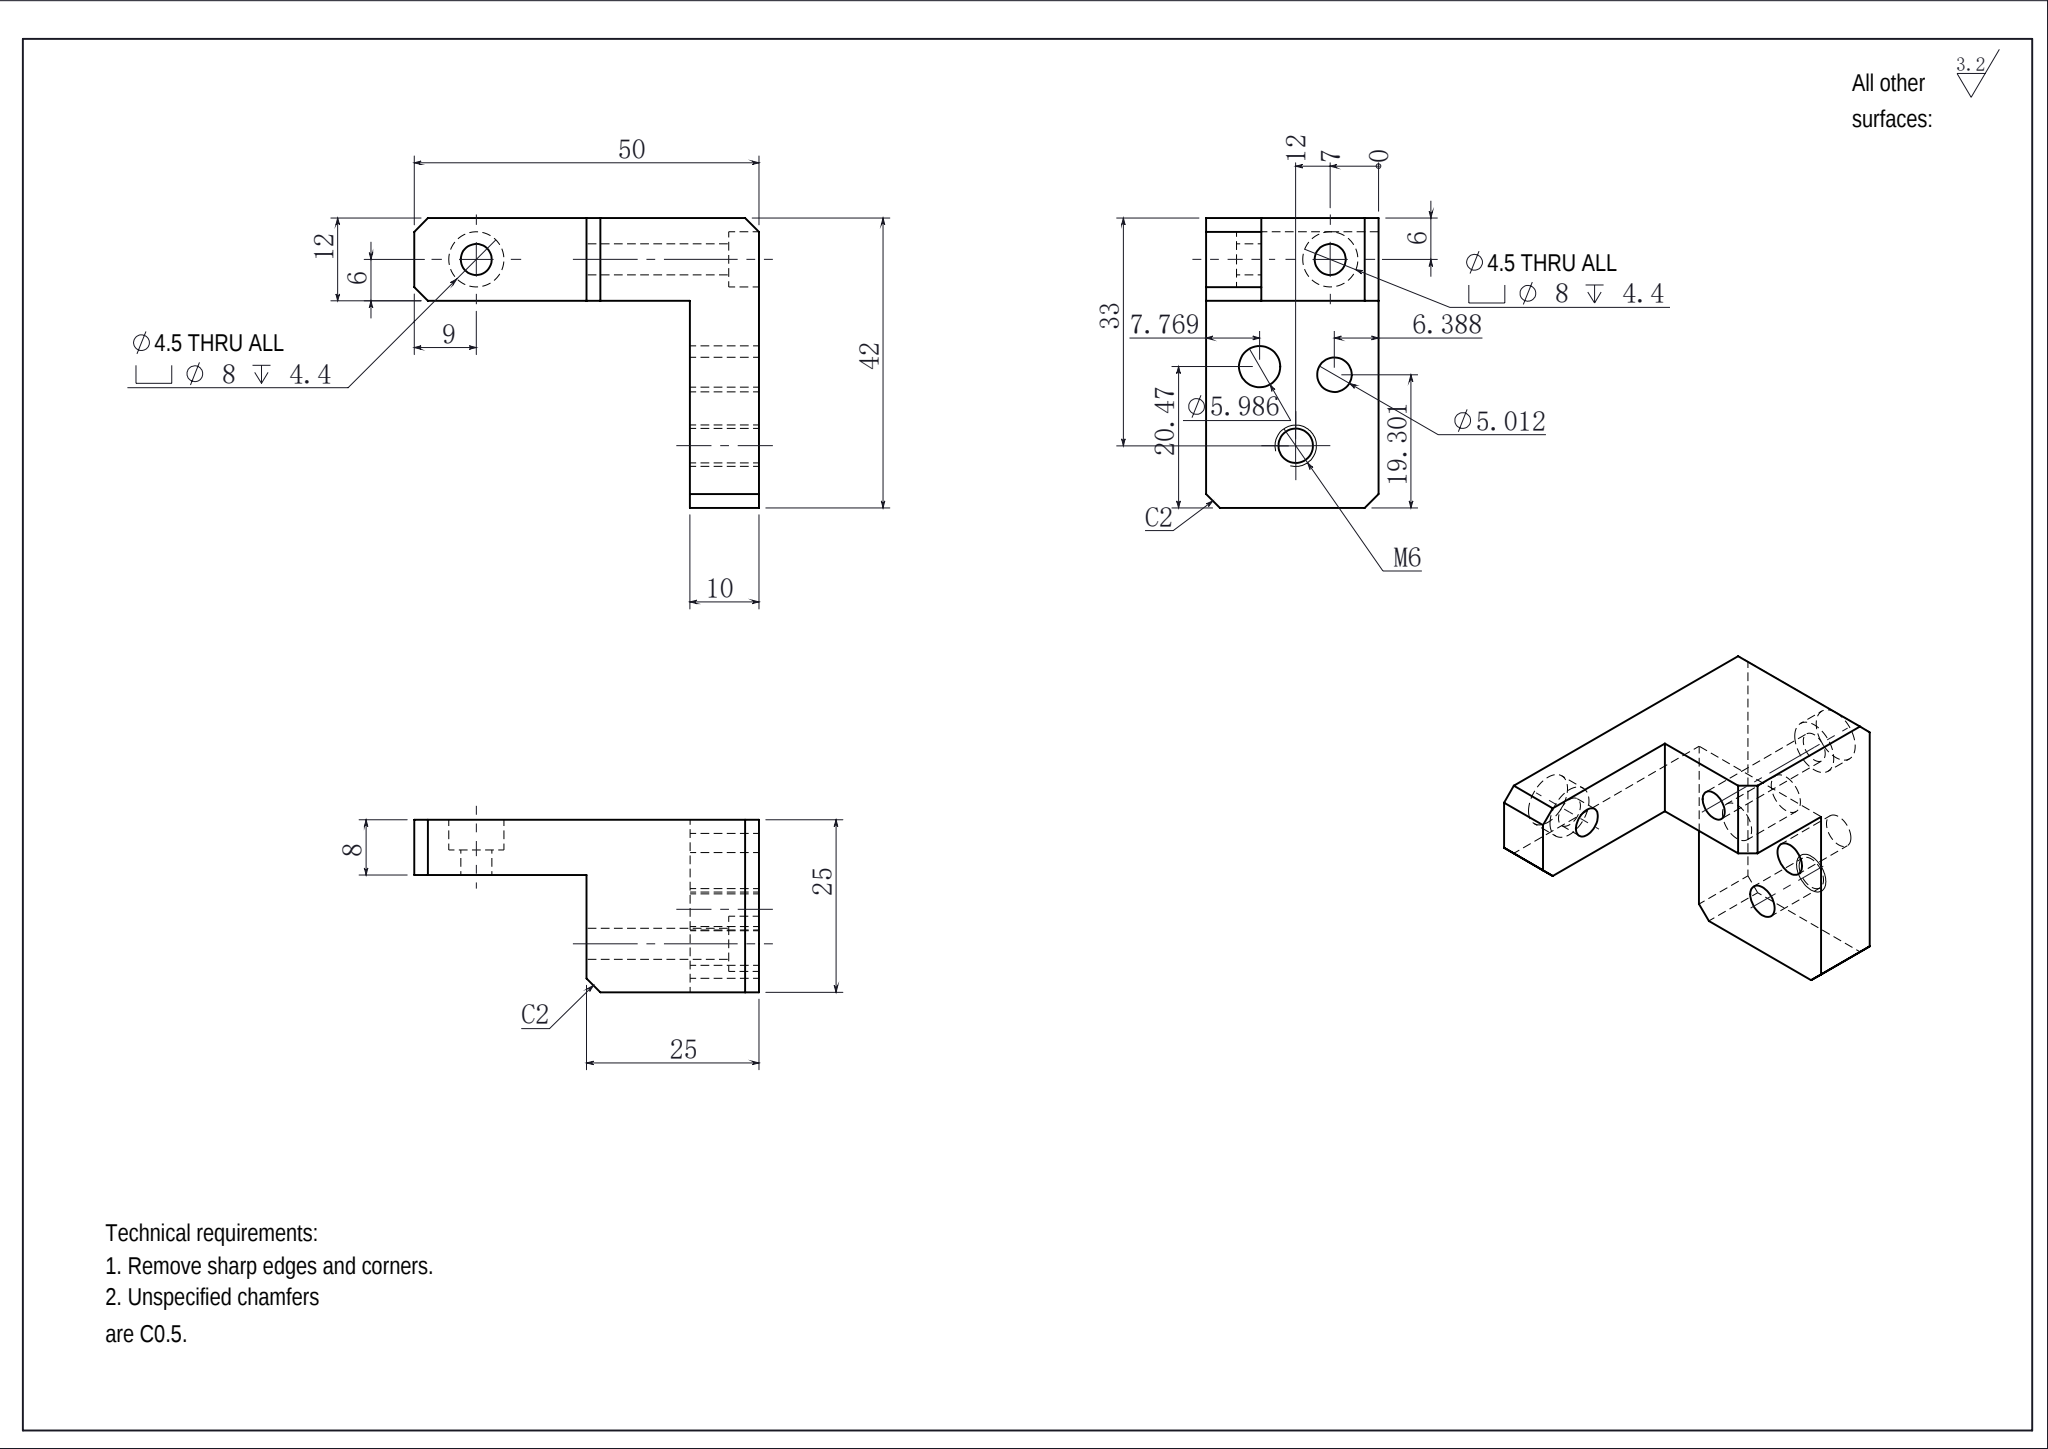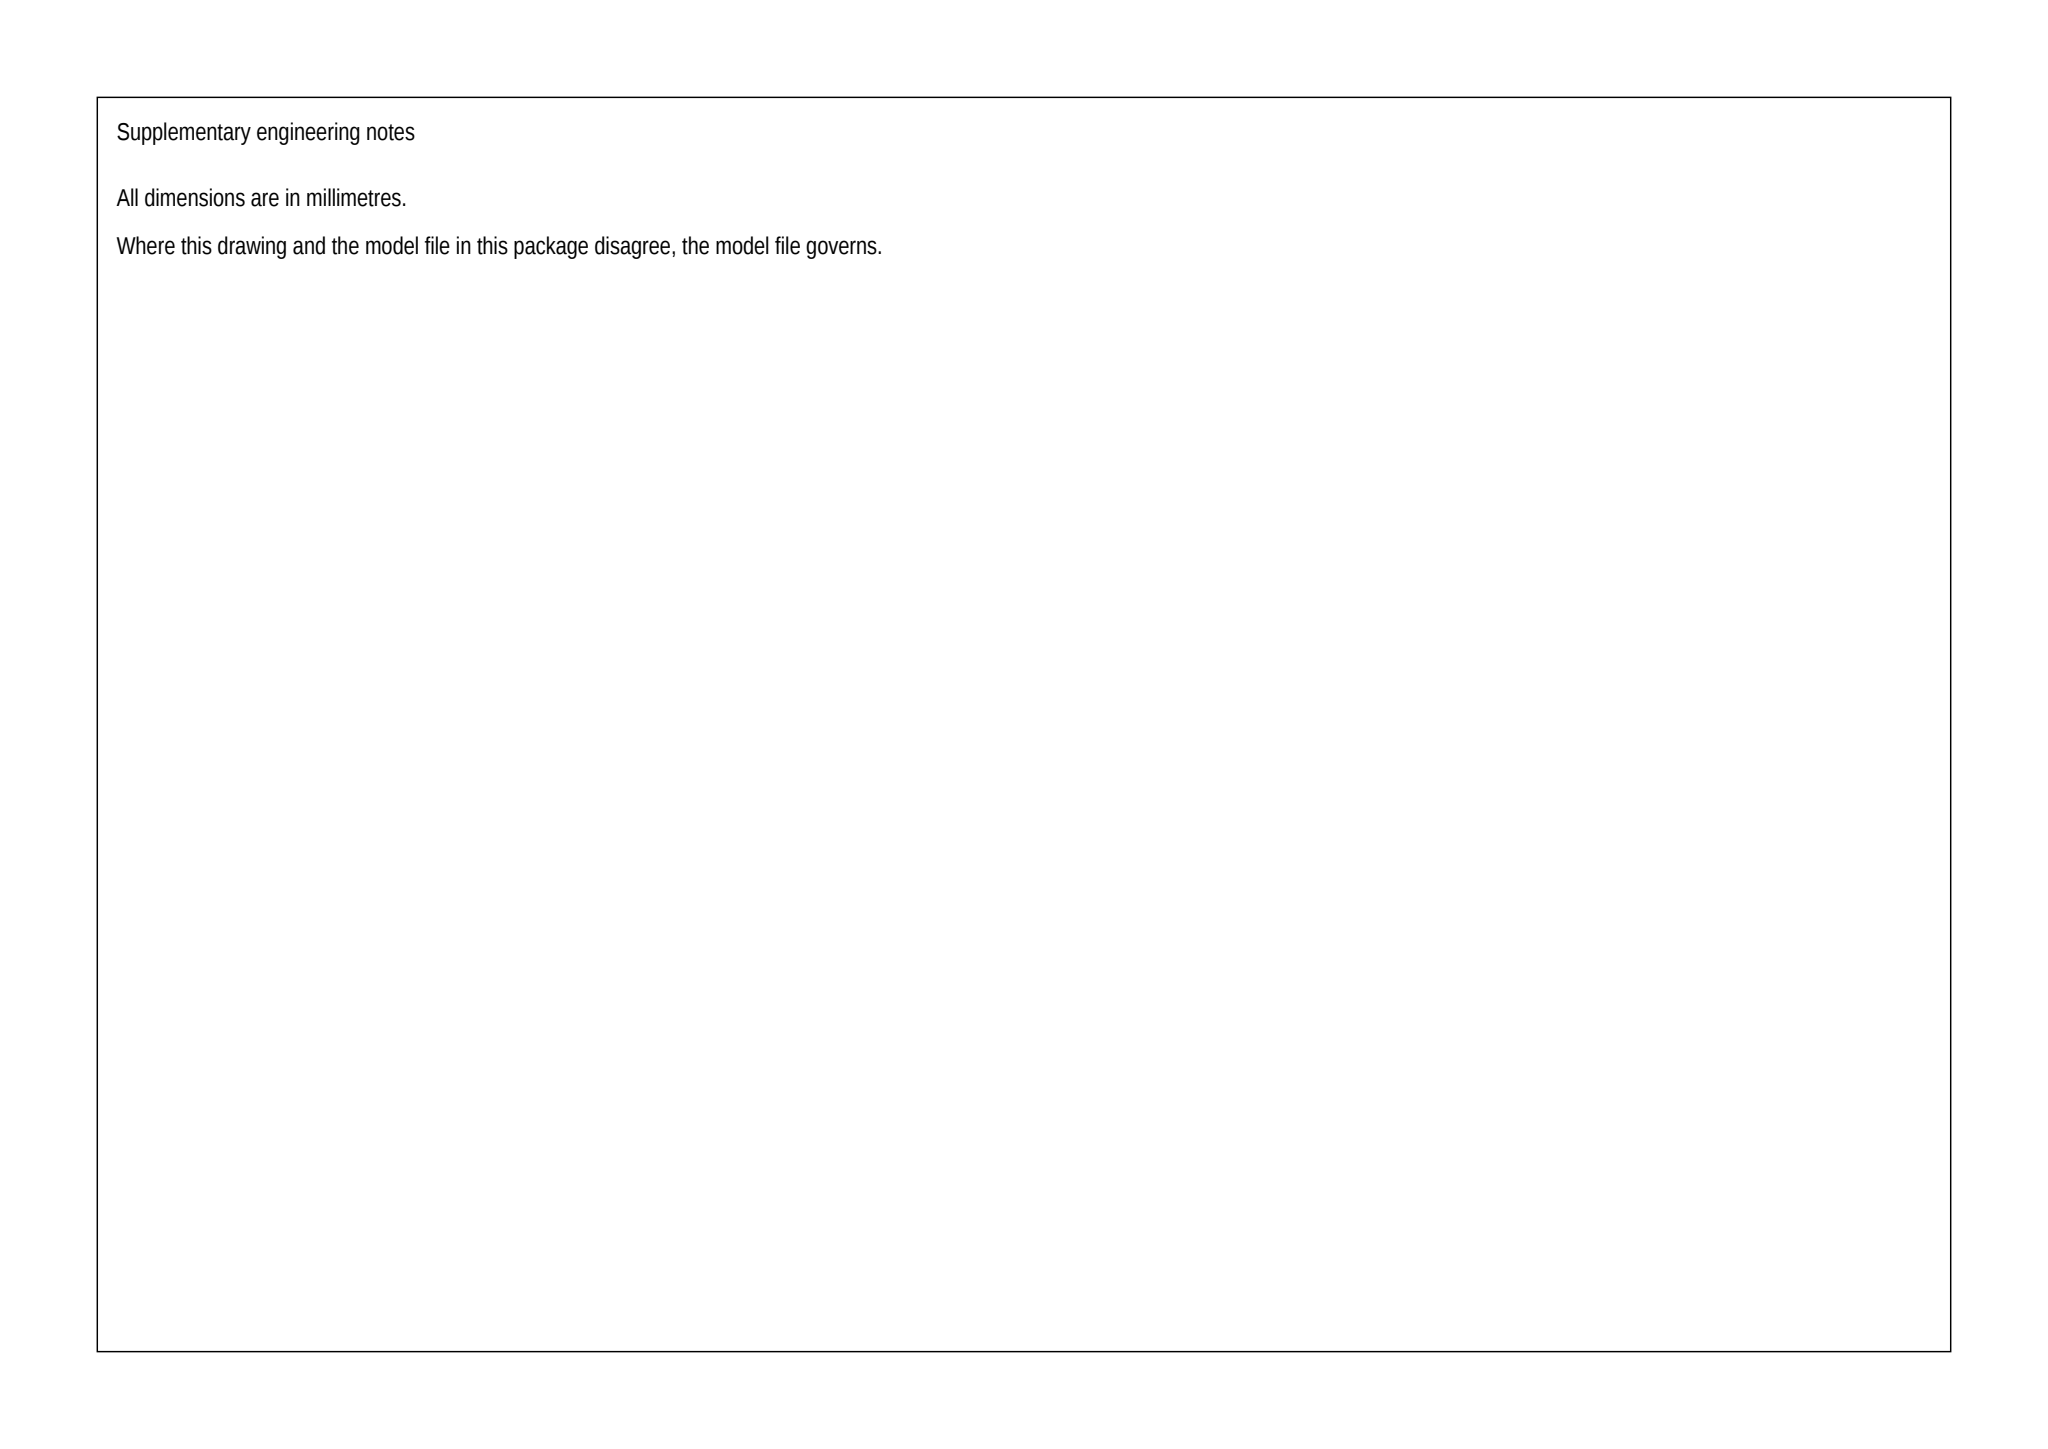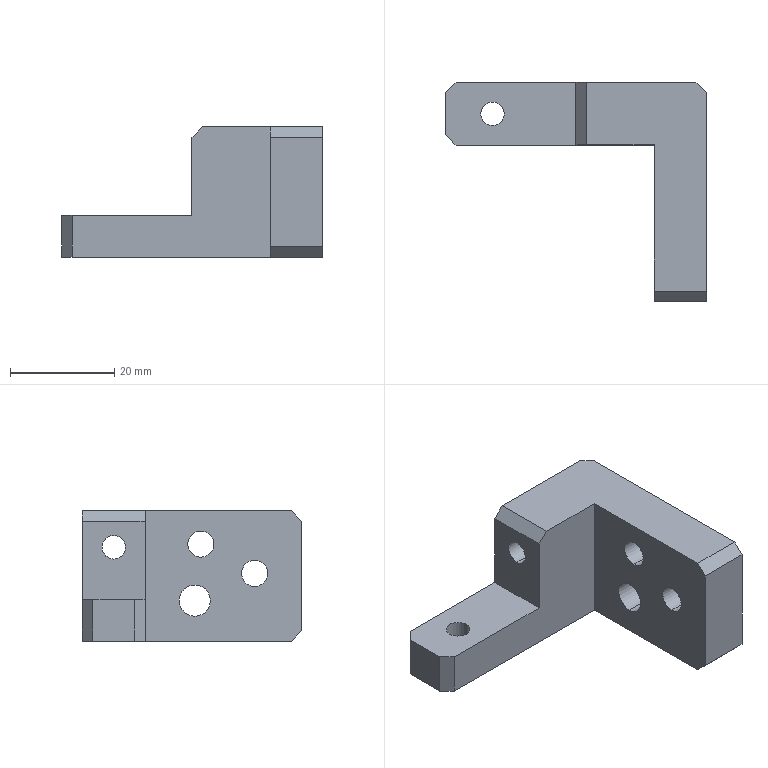Part | SolidWorks | mm | 1 solid | 32 faces | box 50 x 42 x 25 mm | volume 15752 mm3 | plane 18 | cylinder 14 | commonest cylinder face diameters 8 x4 4.5 x4 5.012 x2 5.986 x2 5 x2